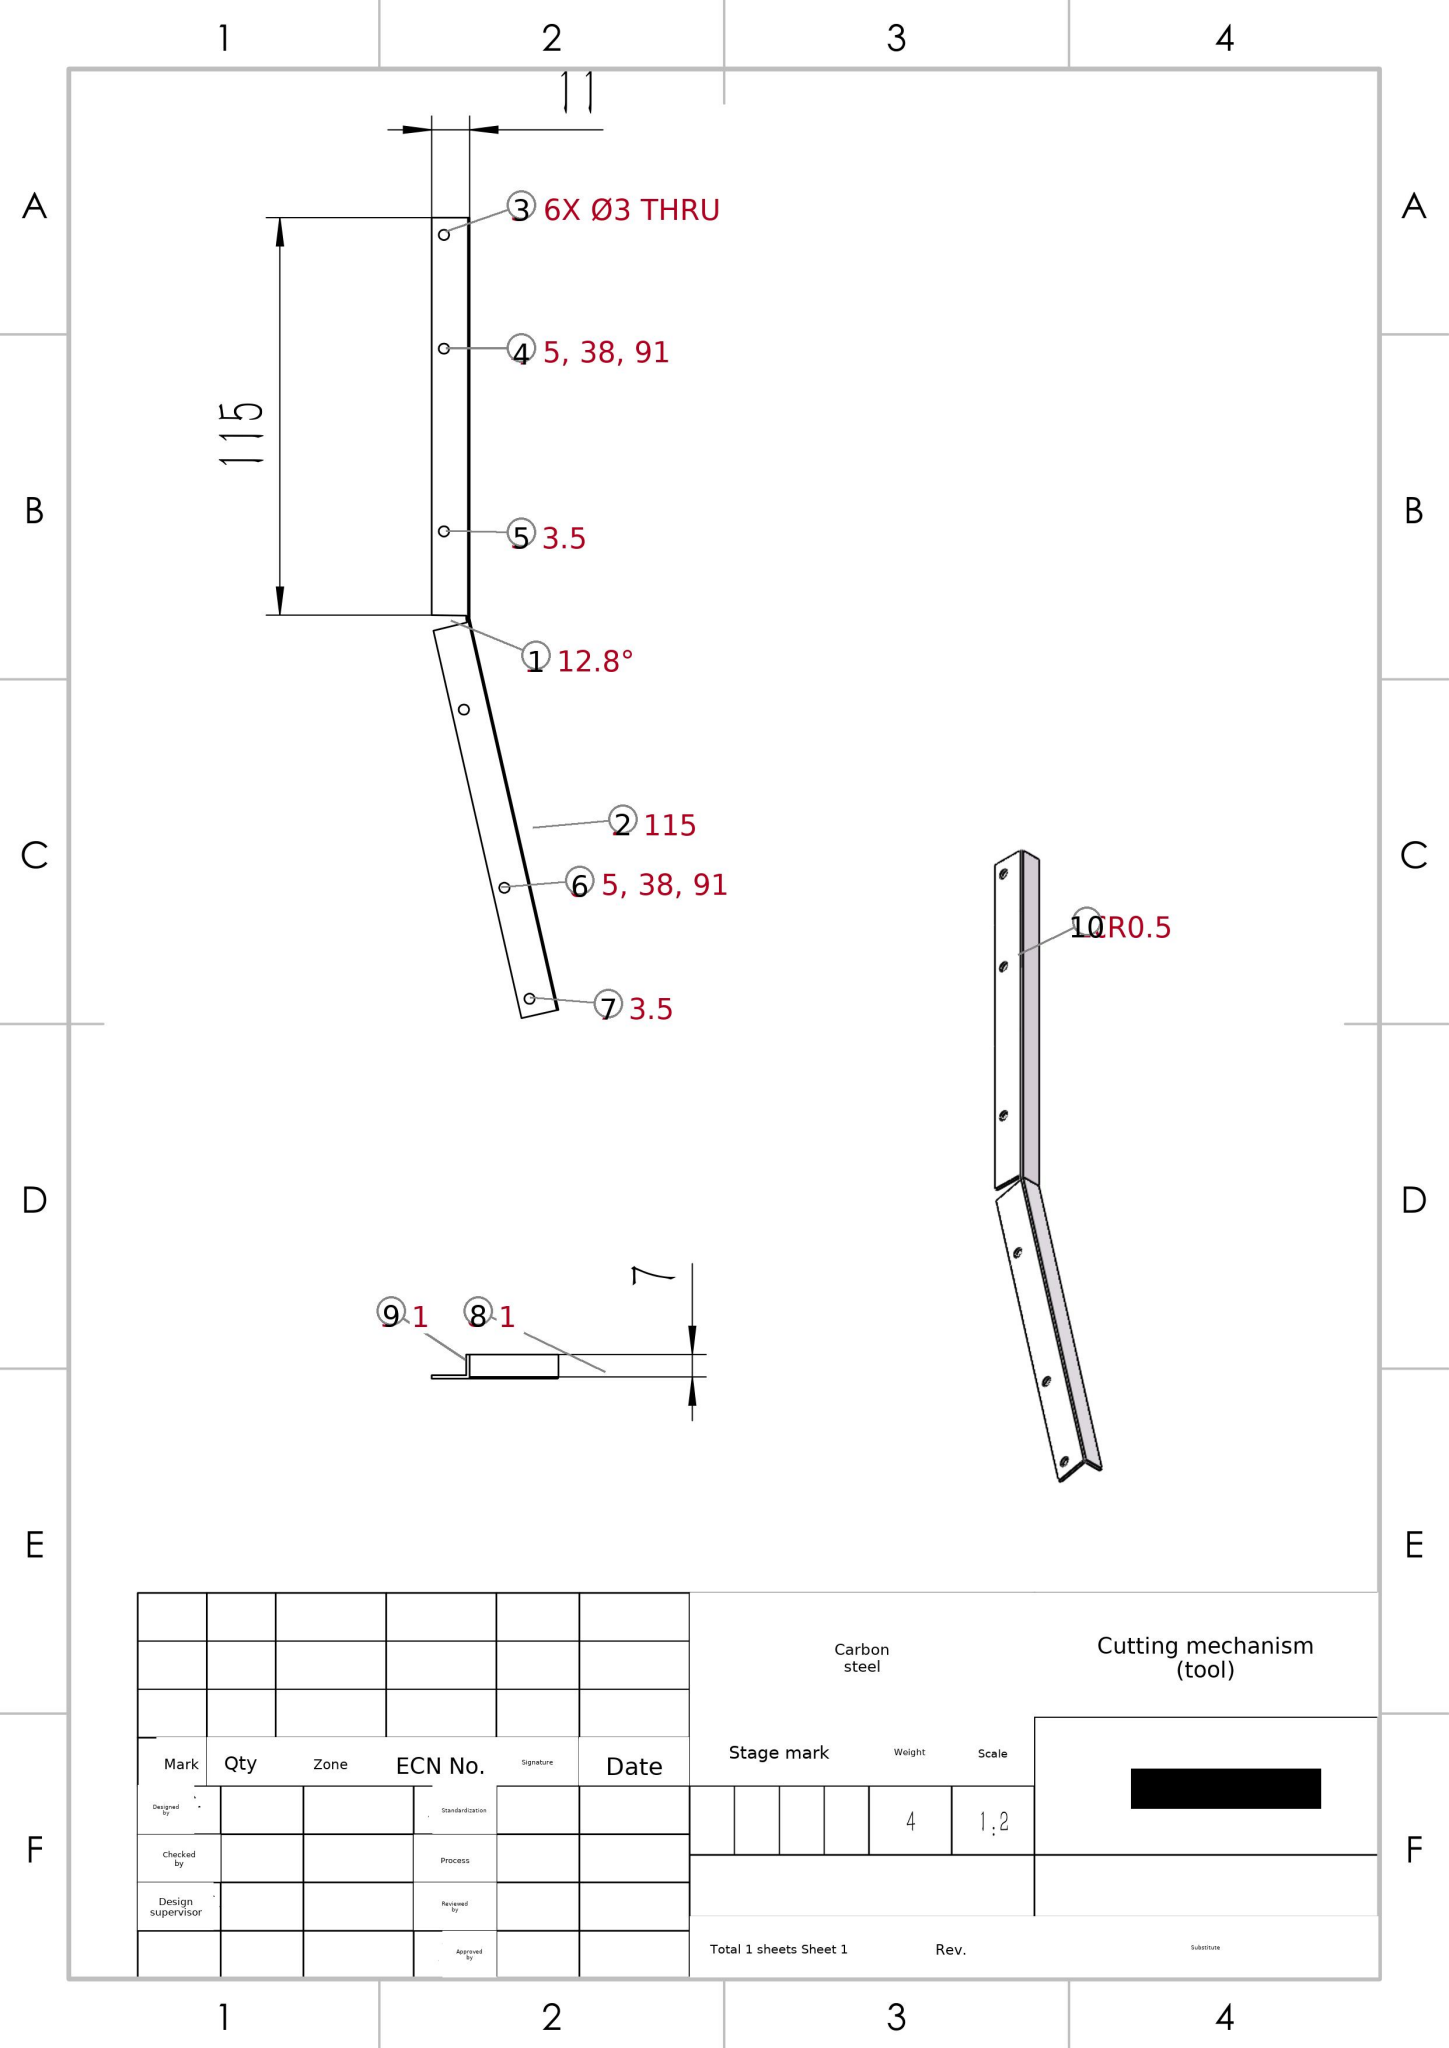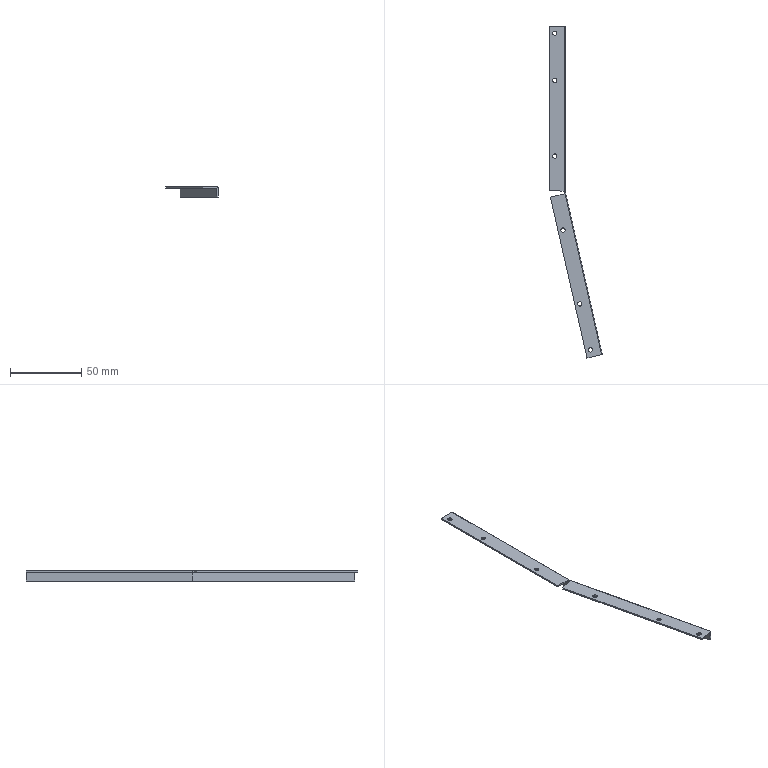Part | SolidWorks | mm | material Carbon steel | 1 solid | 28 faces | box 36.75 x 232.22 x 7 mm | volume 3882 mm3 | plane 14 | cylinder 14 | commonest cylinder face diameters 3 x12 1 x2
STEP:
#1=CARTESIAN_POINT('',(-10.,1.143,0.));
#2=VERTEX_POINT('',#1);
#3=CARTESIAN_POINT('',(0.,1.,0.));
#4=VERTEX_POINT('',#3);
#5=CARTESIAN_POINT('',(0.2085,0.997,-0.));
#6=DIRECTION('',(0.9999,-0.01434,-0.));
#7=VECTOR('',#6,1000.);
#8=LINE('',#5,#7);
#9=EDGE_CURVE('',#2,#4,#8,.T.);
#10=ORIENTED_EDGE('',*,*,#9,.T.);
#11=CARTESIAN_POINT('',(0.,1.,1.));
#12=VERTEX_POINT('',#11);
#13=CARTESIAN_POINT('',(0.,1.,-9.));
#14=DIRECTION('',(0.,0.,1.));
#15=VECTOR('',#14,1000.);
#16=LINE('',#13,#15);
#17=EDGE_CURVE('',#4,#12,#16,.T.);
#18=ORIENTED_EDGE('',*,*,#17,.T.);
#19=CARTESIAN_POINT('',(-10.,1.143,1.));
#20=VERTEX_POINT('',#19);
#21=CARTESIAN_POINT('',(0.01434,0.9998,1.));
#22=DIRECTION('',(-0.9999,0.01434,0.));
#23=VECTOR('',#22,1000.);
#24=LINE('',#21,#23);
#25=EDGE_CURVE('',#12,#20,#24,.T.);
#26=ORIENTED_EDGE('',*,*,#25,.T.);
#27=CARTESIAN_POINT('',(-10.,1.143,0.));
#28=DIRECTION('',(0.,0.,-1.));
#29=VECTOR('',#28,1000.);
#30=LINE('',#27,#29);
#31=EDGE_CURVE('',#20,#2,#30,.T.);
#32=ORIENTED_EDGE('',*,*,#31,.T.);
#33=EDGE_LOOP('',(#10,#18,#26,#32));
#34=FACE_OUTER_BOUND('',#33,.T.);
#35=CARTESIAN_POINT('',(0.01434,0.9998,-9.));
#36=DIRECTION('',(0.01434,0.9999,0.));
#37=DIRECTION('',(0.,0.,-1.));
#38=AXIS2_PLACEMENT_3D('',#35,#36,#37);
#39=PLANE('',#38);
#40=ADVANCED_FACE('',(#34),#39,.F.);
#41=CARTESIAN_POINT('',(-9.499,-3.329,1.));
#42=VERTEX_POINT('',#41);
#43=CARTESIAN_POINT('',(0.2214,-0.9752,1.));
#44=VERTEX_POINT('',#43);
#45=CARTESIAN_POINT('',(-12.308,-4.009,1.));
#46=DIRECTION('',(0.9719,0.2353,0.));
#47=VECTOR('',#46,1000.);
#48=LINE('',#45,#47);
#49=EDGE_CURVE('',#42,#44,#48,.T.);
#50=ORIENTED_EDGE('',*,*,#49,.T.);
#51=CARTESIAN_POINT('',(0.2214,-0.9752,0.));
#52=VERTEX_POINT('',#51);
#53=CARTESIAN_POINT('',(0.2214,-0.9752,-9.));
#54=DIRECTION('',(0.,0.,1.));
#55=VECTOR('',#54,1000.);
#56=LINE('',#53,#55);
#57=EDGE_CURVE('',#52,#44,#56,.T.);
#58=ORIENTED_EDGE('',*,*,#57,.F.);
#59=CARTESIAN_POINT('',(-9.499,-3.329,0.));
#60=VERTEX_POINT('',#59);
#61=CARTESIAN_POINT('',(-2.862,-1.722,0.));
#62=DIRECTION('',(-0.9719,-0.2353,0.));
#63=VECTOR('',#62,1000.);
#64=LINE('',#61,#63);
#65=EDGE_CURVE('',#52,#60,#64,.T.);
#66=ORIENTED_EDGE('',*,*,#65,.T.);
#67=CARTESIAN_POINT('',(-9.499,-3.329,0.));
#68=DIRECTION('',(0.,0.,-1.));
#69=VECTOR('',#68,1000.);
#70=LINE('',#67,#69);
#71=EDGE_CURVE('',#42,#60,#70,.T.);
#72=ORIENTED_EDGE('',*,*,#71,.F.);
#73=EDGE_LOOP('',(#50,#58,#66,#72));
#74=FACE_OUTER_BOUND('',#73,.T.);
#75=CARTESIAN_POINT('',(0.2353,-0.9718,-9.));
#76=DIRECTION('',(0.2353,-0.9719,0.));
#77=DIRECTION('',(0.,0.,-1.));
#78=AXIS2_PLACEMENT_3D('',#75,#76,#77);
#79=PLANE('',#78);
#80=ADVANCED_FACE('',(#74),#79,.F.);
#81=CARTESIAN_POINT('',(-7.96,25.45,0.));
#82=VERTEX_POINT('',#81);
#83=CARTESIAN_POINT('',(-7.96,25.45,1.));
#84=VERTEX_POINT('',#83);
#85=CARTESIAN_POINT('',(-7.96,25.45,-9.));
#86=DIRECTION('',(0.,0.,1.));
#87=VECTOR('',#86,1000.);
#88=LINE('',#85,#87);
#89=EDGE_CURVE('',#82,#84,#88,.T.);
#90=ORIENTED_EDGE('',*,*,#89,.F.);
#91=CARTESIAN_POINT('',(-4.96,25.45,-0.));
#92=VERTEX_POINT('',#91);
#93=CARTESIAN_POINT('',(-6.46,25.45,0.));
#94=DIRECTION('',(-0.,-0.,-1.));
#95=DIRECTION('',(-1.,0.,0.));
#96=AXIS2_PLACEMENT_3D('',#93,#94,#95);
#97=CIRCLE('',#96,1.5);
#98=EDGE_CURVE('',#82,#92,#97,.T.);
#99=ORIENTED_EDGE('',*,*,#98,.T.);
#100=CARTESIAN_POINT('',(-4.96,25.45,1.));
#101=VERTEX_POINT('',#100);
#102=CARTESIAN_POINT('',(-4.96,25.45,-9.));
#103=DIRECTION('',(0.,0.,1.));
#104=VECTOR('',#103,1000.);
#105=LINE('',#102,#104);
#106=EDGE_CURVE('',#92,#101,#105,.T.);
#107=ORIENTED_EDGE('',*,*,#106,.T.);
#108=CARTESIAN_POINT('',(-6.46,25.45,1.));
#109=DIRECTION('',(0.,0.,1.));
#110=DIRECTION('',(1.,0.,0.));
#111=AXIS2_PLACEMENT_3D('',#108,#109,#110);
#112=CIRCLE('',#111,1.5);
#113=EDGE_CURVE('',#101,#84,#112,.T.);
#114=ORIENTED_EDGE('',*,*,#113,.T.);
#115=EDGE_LOOP('',(#90,#99,#107,#114));
#116=FACE_OUTER_BOUND('',#115,.T.);
#117=CARTESIAN_POINT('',(-6.46,25.45,-9.));
#118=DIRECTION('',(0.,0.,1.));
#119=DIRECTION('',(1.,0.,0.));
#120=AXIS2_PLACEMENT_3D('',#117,#118,#119);
#121=CYLINDRICAL_SURFACE('',#120,1.5);
#122=ADVANCED_FACE('',(#116),#121,.F.);
#123=CARTESIAN_POINT('',(16.871,-110.115,-0.));
#124=VERTEX_POINT('',#123);
#125=CARTESIAN_POINT('',(16.871,-110.115,1.));
#126=VERTEX_POINT('',#125);
#127=CARTESIAN_POINT('',(16.871,-110.115,-9.));
#128=DIRECTION('',(0.,0.,1.));
#129=VECTOR('',#128,1000.);
#130=LINE('',#127,#129);
#131=EDGE_CURVE('',#124,#126,#130,.T.);
#132=ORIENTED_EDGE('',*,*,#131,.F.);
#133=CARTESIAN_POINT('',(19.871,-110.115,-0.));
#134=VERTEX_POINT('',#133);
#135=CARTESIAN_POINT('',(18.371,-110.115,-0.));
#136=DIRECTION('',(-0.,-0.,-1.));
#137=DIRECTION('',(-1.,0.,0.));
#138=AXIS2_PLACEMENT_3D('',#135,#136,#137);
#139=CIRCLE('',#138,1.5);
#140=EDGE_CURVE('',#124,#134,#139,.T.);
#141=ORIENTED_EDGE('',*,*,#140,.T.);
#142=CARTESIAN_POINT('',(19.871,-110.115,1.));
#143=VERTEX_POINT('',#142);
#144=CARTESIAN_POINT('',(19.871,-110.115,-9.));
#145=DIRECTION('',(0.,0.,1.));
#146=VECTOR('',#145,1000.);
#147=LINE('',#144,#146);
#148=EDGE_CURVE('',#134,#143,#147,.T.);
#149=ORIENTED_EDGE('',*,*,#148,.T.);
#150=CARTESIAN_POINT('',(18.371,-110.115,1.));
#151=DIRECTION('',(0.,0.,1.));
#152=DIRECTION('',(-1.,0.,0.));
#153=AXIS2_PLACEMENT_3D('',#150,#151,#152);
#154=CIRCLE('',#153,1.5);
#155=EDGE_CURVE('',#143,#126,#154,.T.);
#156=ORIENTED_EDGE('',*,*,#155,.T.);
#157=EDGE_LOOP('',(#132,#141,#149,#156));
#158=FACE_OUTER_BOUND('',#157,.T.);
#159=CARTESIAN_POINT('',(18.371,-110.115,-9.));
#160=DIRECTION('',(0.,0.,1.));
#161=DIRECTION('',(1.,0.,0.));
#162=AXIS2_PLACEMENT_3D('',#159,#160,#161);
#163=CYLINDRICAL_SURFACE('',#162,1.5);
#164=ADVANCED_FACE('',(#158),#163,.F.);
#165=CARTESIAN_POINT('',(9.566,-77.934,-0.));
#166=VERTEX_POINT('',#165);
#167=CARTESIAN_POINT('',(9.566,-77.934,1.));
#168=VERTEX_POINT('',#167);
#169=CARTESIAN_POINT('',(9.566,-77.934,-9.));
#170=DIRECTION('',(0.,0.,1.));
#171=VECTOR('',#170,1000.);
#172=LINE('',#169,#171);
#173=EDGE_CURVE('',#166,#168,#172,.T.);
#174=ORIENTED_EDGE('',*,*,#173,.F.);
#175=CARTESIAN_POINT('',(12.566,-77.934,-0.));
#176=VERTEX_POINT('',#175);
#177=CARTESIAN_POINT('',(11.066,-77.934,-0.));
#178=DIRECTION('',(-0.,-0.,-1.));
#179=DIRECTION('',(-1.,0.,0.));
#180=AXIS2_PLACEMENT_3D('',#177,#178,#179);
#181=CIRCLE('',#180,1.5);
#182=EDGE_CURVE('',#166,#176,#181,.T.);
#183=ORIENTED_EDGE('',*,*,#182,.T.);
#184=CARTESIAN_POINT('',(12.566,-77.934,1.));
#185=VERTEX_POINT('',#184);
#186=CARTESIAN_POINT('',(12.566,-77.934,-9.));
#187=DIRECTION('',(0.,0.,1.));
#188=VECTOR('',#187,1000.);
#189=LINE('',#186,#188);
#190=EDGE_CURVE('',#176,#185,#189,.T.);
#191=ORIENTED_EDGE('',*,*,#190,.T.);
#192=CARTESIAN_POINT('',(11.066,-77.934,1.));
#193=DIRECTION('',(0.,0.,1.));
#194=DIRECTION('',(-1.,0.,0.));
#195=AXIS2_PLACEMENT_3D('',#192,#193,#194);
#196=CIRCLE('',#195,1.5);
#197=EDGE_CURVE('',#185,#168,#196,.T.);
#198=ORIENTED_EDGE('',*,*,#197,.T.);
#199=EDGE_LOOP('',(#174,#183,#191,#198));
#200=FACE_OUTER_BOUND('',#199,.T.);
#201=CARTESIAN_POINT('',(11.066,-77.934,-9.));
#202=DIRECTION('',(0.,0.,1.));
#203=DIRECTION('',(1.,0.,0.));
#204=AXIS2_PLACEMENT_3D('',#201,#202,#203);
#205=CYLINDRICAL_SURFACE('',#204,1.5);
#206=ADVANCED_FACE('',(#200),#205,.F.);
#207=CARTESIAN_POINT('',(-2.166,-26.249,0.));
#208=VERTEX_POINT('',#207);
#209=CARTESIAN_POINT('',(-2.166,-26.249,1.));
#210=VERTEX_POINT('',#209);
#211=CARTESIAN_POINT('',(-2.166,-26.249,-9.));
#212=DIRECTION('',(0.,0.,1.));
#213=VECTOR('',#212,1000.);
#214=LINE('',#211,#213);
#215=EDGE_CURVE('',#208,#210,#214,.T.);
#216=ORIENTED_EDGE('',*,*,#215,.F.);
#217=CARTESIAN_POINT('',(0.8338,-26.249,-0.));
#218=VERTEX_POINT('',#217);
#219=CARTESIAN_POINT('',(-0.6662,-26.249,0.));
#220=DIRECTION('',(-0.,-0.,-1.));
#221=DIRECTION('',(-1.,0.,0.));
#222=AXIS2_PLACEMENT_3D('',#219,#220,#221);
#223=CIRCLE('',#222,1.5);
#224=EDGE_CURVE('',#208,#218,#223,.T.);
#225=ORIENTED_EDGE('',*,*,#224,.T.);
#226=CARTESIAN_POINT('',(0.8338,-26.249,1.));
#227=VERTEX_POINT('',#226);
#228=CARTESIAN_POINT('',(0.8338,-26.249,-9.));
#229=DIRECTION('',(0.,0.,1.));
#230=VECTOR('',#229,1000.);
#231=LINE('',#228,#230);
#232=EDGE_CURVE('',#218,#227,#231,.T.);
#233=ORIENTED_EDGE('',*,*,#232,.T.);
#234=CARTESIAN_POINT('',(-0.6662,-26.249,1.));
#235=DIRECTION('',(0.,0.,1.));
#236=DIRECTION('',(-1.,0.,0.));
#237=AXIS2_PLACEMENT_3D('',#234,#235,#236);
#238=CIRCLE('',#237,1.5);
#239=EDGE_CURVE('',#227,#210,#238,.T.);
#240=ORIENTED_EDGE('',*,*,#239,.T.);
#241=EDGE_LOOP('',(#216,#225,#233,#240));
#242=FACE_OUTER_BOUND('',#241,.T.);
#243=CARTESIAN_POINT('',(-0.6662,-26.249,-9.));
#244=DIRECTION('',(0.,0.,1.));
#245=DIRECTION('',(1.,0.,0.));
#246=AXIS2_PLACEMENT_3D('',#243,#244,#245);
#247=CYLINDRICAL_SURFACE('',#246,1.5);
#248=ADVANCED_FACE('',(#242),#247,.F.);
#249=CARTESIAN_POINT('',(-7.96,78.45,0.));
#250=VERTEX_POINT('',#249);
#251=CARTESIAN_POINT('',(-7.96,78.45,1.));
#252=VERTEX_POINT('',#251);
#253=CARTESIAN_POINT('',(-7.96,78.45,-9.));
#254=DIRECTION('',(0.,0.,1.));
#255=VECTOR('',#254,1000.);
#256=LINE('',#253,#255);
#257=EDGE_CURVE('',#250,#252,#256,.T.);
#258=ORIENTED_EDGE('',*,*,#257,.F.);
#259=CARTESIAN_POINT('',(-4.96,78.45,-0.));
#260=VERTEX_POINT('',#259);
#261=CARTESIAN_POINT('',(-6.46,78.45,0.));
#262=DIRECTION('',(-0.,-0.,-1.));
#263=DIRECTION('',(-1.,0.,0.));
#264=AXIS2_PLACEMENT_3D('',#261,#262,#263);
#265=CIRCLE('',#264,1.5);
#266=EDGE_CURVE('',#250,#260,#265,.T.);
#267=ORIENTED_EDGE('',*,*,#266,.T.);
#268=CARTESIAN_POINT('',(-4.96,78.45,1.));
#269=VERTEX_POINT('',#268);
#270=CARTESIAN_POINT('',(-4.96,78.45,-9.));
#271=DIRECTION('',(0.,0.,1.));
#272=VECTOR('',#271,1000.);
#273=LINE('',#270,#272);
#274=EDGE_CURVE('',#260,#269,#273,.T.);
#275=ORIENTED_EDGE('',*,*,#274,.T.);
#276=CARTESIAN_POINT('',(-6.46,78.45,1.));
#277=DIRECTION('',(0.,0.,1.));
#278=DIRECTION('',(1.,0.,0.));
#279=AXIS2_PLACEMENT_3D('',#276,#277,#278);
#280=CIRCLE('',#279,1.5);
#281=EDGE_CURVE('',#269,#252,#280,.T.);
#282=ORIENTED_EDGE('',*,*,#281,.T.);
#283=EDGE_LOOP('',(#258,#267,#275,#282));
#284=FACE_OUTER_BOUND('',#283,.T.);
#285=CARTESIAN_POINT('',(-6.46,78.45,-9.));
#286=DIRECTION('',(0.,0.,1.));
#287=DIRECTION('',(1.,0.,0.));
#288=AXIS2_PLACEMENT_3D('',#285,#286,#287);
#289=CYLINDRICAL_SURFACE('',#288,1.5);
#290=ADVANCED_FACE('',(#284),#289,.F.);
#291=CARTESIAN_POINT('',(-7.96,111.45,0.));
#292=VERTEX_POINT('',#291);
#293=CARTESIAN_POINT('',(-7.96,111.45,1.));
#294=VERTEX_POINT('',#293);
#295=CARTESIAN_POINT('',(-7.96,111.45,-9.));
#296=DIRECTION('',(0.,0.,1.));
#297=VECTOR('',#296,1000.);
#298=LINE('',#295,#297);
#299=EDGE_CURVE('',#292,#294,#298,.T.);
#300=ORIENTED_EDGE('',*,*,#299,.F.);
#301=CARTESIAN_POINT('',(-4.96,111.45,-0.));
#302=VERTEX_POINT('',#301);
#303=CARTESIAN_POINT('',(-6.46,111.45,0.));
#304=DIRECTION('',(-0.,-0.,-1.));
#305=DIRECTION('',(-1.,0.,0.));
#306=AXIS2_PLACEMENT_3D('',#303,#304,#305);
#307=CIRCLE('',#306,1.5);
#308=EDGE_CURVE('',#292,#302,#307,.T.);
#309=ORIENTED_EDGE('',*,*,#308,.T.);
#310=CARTESIAN_POINT('',(-4.96,111.45,1.));
#311=VERTEX_POINT('',#310);
#312=CARTESIAN_POINT('',(-4.96,111.45,-9.));
#313=DIRECTION('',(0.,0.,1.));
#314=VECTOR('',#313,1000.);
#315=LINE('',#312,#314);
#316=EDGE_CURVE('',#302,#311,#315,.T.);
#317=ORIENTED_EDGE('',*,*,#316,.T.);
#318=CARTESIAN_POINT('',(-6.46,111.45,1.));
#319=DIRECTION('',(0.,0.,1.));
#320=DIRECTION('',(1.,0.,0.));
#321=AXIS2_PLACEMENT_3D('',#318,#319,#320);
#322=CIRCLE('',#321,1.5);
#323=EDGE_CURVE('',#311,#294,#322,.T.);
#324=ORIENTED_EDGE('',*,*,#323,.T.);
#325=EDGE_LOOP('',(#300,#309,#317,#324));
#326=FACE_OUTER_BOUND('',#325,.T.);
#327=CARTESIAN_POINT('',(-6.46,111.45,-9.));
#328=DIRECTION('',(0.,0.,1.));
#329=DIRECTION('',(1.,0.,0.));
#330=AXIS2_PLACEMENT_3D('',#327,#328,#329);
#331=CYLINDRICAL_SURFACE('',#330,1.5);
#332=ADVANCED_FACE('',(#326),#331,.F.);
#333=CARTESIAN_POINT('',(26.752,-113.34,0.5));
#334=VERTEX_POINT('',#333);
#335=CARTESIAN_POINT('',(26.265,-113.451,1.));
#336=VERTEX_POINT('',#335);
#337=CARTESIAN_POINT('',(26.265,-113.451,0.5));
#338=DIRECTION('',(0.2214,-0.9752,0.));
#339=DIRECTION('',(0.9752,0.2214,0.));
#340=AXIS2_PLACEMENT_3D('',#337,#338,#339);
#341=CIRCLE('',#340,0.5);
#342=EDGE_CURVE('',#334,#336,#341,.T.);
#343=ORIENTED_EDGE('',*,*,#342,.T.);
#344=CARTESIAN_POINT('',(16.025,-115.775,1.));
#345=VERTEX_POINT('',#344);
#346=CARTESIAN_POINT('',(14.684,-116.079,1.));
#347=DIRECTION('',(-0.9752,-0.2214,0.));
#348=VECTOR('',#347,1000.);
#349=LINE('',#346,#348);
#350=EDGE_CURVE('',#336,#345,#349,.T.);
#351=ORIENTED_EDGE('',*,*,#350,.T.);
#352=CARTESIAN_POINT('',(16.025,-115.775,0.));
#353=VERTEX_POINT('',#352);
#354=CARTESIAN_POINT('',(16.025,-115.775,0.));
#355=DIRECTION('',(0.,0.,-1.));
#356=VECTOR('',#355,1000.);
#357=LINE('',#354,#356);
#358=EDGE_CURVE('',#345,#353,#357,.T.);
#359=ORIENTED_EDGE('',*,*,#358,.T.);
#360=CARTESIAN_POINT('',(25.777,-113.561,0.));
#361=VERTEX_POINT('',#360);
#362=CARTESIAN_POINT('',(24.315,-113.893,0.));
#363=DIRECTION('',(0.9752,0.2214,-0.));
#364=VECTOR('',#363,1000.);
#365=LINE('',#362,#364);
#366=EDGE_CURVE('',#353,#361,#365,.T.);
#367=ORIENTED_EDGE('',*,*,#366,.T.);
#368=CARTESIAN_POINT('',(25.777,-113.561,-6.));
#369=VERTEX_POINT('',#368);
#370=CARTESIAN_POINT('',(25.777,-113.561,-6.));
#371=DIRECTION('',(0.,0.,-1.));
#372=VECTOR('',#371,1000.);
#373=LINE('',#370,#372);
#374=EDGE_CURVE('',#361,#369,#373,.T.);
#375=ORIENTED_EDGE('',*,*,#374,.T.);
#376=CARTESIAN_POINT('',(26.752,-113.34,-6.));
#377=VERTEX_POINT('',#376);
#378=CARTESIAN_POINT('',(25.279,-113.674,-6.));
#379=DIRECTION('',(0.9752,0.2214,0.));
#380=VECTOR('',#379,1000.);
#381=LINE('',#378,#380);
#382=EDGE_CURVE('',#369,#377,#381,.T.);
#383=ORIENTED_EDGE('',*,*,#382,.T.);
#384=CARTESIAN_POINT('',(26.752,-113.34,0.5));
#385=DIRECTION('',(-0.,-0.,1.));
#386=VECTOR('',#385,1000.);
#387=LINE('',#384,#386);
#388=EDGE_CURVE('',#377,#334,#387,.T.);
#389=ORIENTED_EDGE('',*,*,#388,.T.);
#390=EDGE_LOOP('',(#343,#351,#359,#367,#375,#383,#389));
#391=FACE_OUTER_BOUND('',#390,.T.);
#392=CARTESIAN_POINT('',(21.389,-114.557,-2.5));
#393=DIRECTION('',(0.2214,-0.9752,0.));
#394=DIRECTION('',(0.,0.,-1.));
#395=AXIS2_PLACEMENT_3D('',#392,#393,#394);
#396=PLANE('',#395);
#397=ADVANCED_FACE('',(#391),#396,.T.);
#398=CARTESIAN_POINT('',(1.,0.1121,0.5));
#399=VERTEX_POINT('',#398);
#400=CARTESIAN_POINT('',(1.,116.45,0.5));
#401=VERTEX_POINT('',#400);
#402=CARTESIAN_POINT('',(1.,-13.543,0.5));
#403=DIRECTION('',(-0.,1.,0.));
#404=VECTOR('',#403,1000.);
#405=LINE('',#402,#404);
#406=EDGE_CURVE('',#399,#401,#405,.T.);
#407=ORIENTED_EDGE('',*,*,#406,.F.);
#408=CARTESIAN_POINT('',(1.,0.1121,-6.));
#409=VERTEX_POINT('',#408);
#410=CARTESIAN_POINT('',(1.,0.1121,0.5));
#411=DIRECTION('',(0.,0.,-1.));
#412=VECTOR('',#411,1000.);
#413=LINE('',#410,#412);
#414=EDGE_CURVE('',#399,#409,#413,.T.);
#415=ORIENTED_EDGE('',*,*,#414,.T.);
#416=CARTESIAN_POINT('',(1.,116.45,-6.));
#417=VERTEX_POINT('',#416);
#418=CARTESIAN_POINT('',(1.,-13.543,-6.));
#419=DIRECTION('',(-0.,1.,0.));
#420=VECTOR('',#419,1000.);
#421=LINE('',#418,#420);
#422=EDGE_CURVE('',#409,#417,#421,.T.);
#423=ORIENTED_EDGE('',*,*,#422,.T.);
#424=CARTESIAN_POINT('',(1.,116.45,0.5));
#425=DIRECTION('',(0.,0.,-1.));
#426=VECTOR('',#425,1000.);
#427=LINE('',#424,#426);
#428=EDGE_CURVE('',#401,#417,#427,.T.);
#429=ORIENTED_EDGE('',*,*,#428,.F.);
#430=EDGE_LOOP('',(#407,#415,#423,#429));
#431=FACE_OUTER_BOUND('',#430,.T.);
#432=CARTESIAN_POINT('',(1.,-13.543,0.5));
#433=DIRECTION('',(1.,0.,0.));
#434=DIRECTION('',(-0.,0.,1.));
#435=AXIS2_PLACEMENT_3D('',#432,#433,#434);
#436=PLANE('',#435);
#437=ADVANCED_FACE('',(#431),#436,.T.);
#438=CARTESIAN_POINT('',(0.5,0.05603,1.));
#439=VERTEX_POINT('',#438);
#440=CARTESIAN_POINT('',(0.5,116.45,1.));
#441=VERTEX_POINT('',#440);
#442=CARTESIAN_POINT('',(0.5,-13.543,1.));
#443=DIRECTION('',(-0.,1.,0.));
#444=VECTOR('',#443,1000.);
#445=LINE('',#442,#444);
#446=EDGE_CURVE('',#439,#441,#445,.T.);
#447=ORIENTED_EDGE('',*,*,#446,.F.);
#448=CARTESIAN_POINT('',(0.5,0.05603,1.));
#449=CARTESIAN_POINT('',(0.7929,0.08886,1.));
#450=CARTESIAN_POINT('',(1.,0.1121,0.7929));
#451=CARTESIAN_POINT('',(1.,0.1121,0.5));
#452=(BOUNDED_CURVE()B_SPLINE_CURVE(3,(#448,#449,#450,#451),.UNSPECIFIED.,.F.,.F.)B_SPLINE_CURVE_WITH_KNOTS((4,4),(4.712,6.283),.UNSPECIFIED.)CURVE()GEOMETRIC_REPRESENTATION_ITEM()RATIONAL_B_SPLINE_CURVE((1.,0.8047,0.8047,1.))REPRESENTATION_ITEM(''));
#453=EDGE_CURVE('',#439,#399,#452,.T.);
#454=ORIENTED_EDGE('',*,*,#453,.T.);
#455=ORIENTED_EDGE('',*,*,#406,.T.);
#456=CARTESIAN_POINT('',(0.5,116.45,0.5));
#457=DIRECTION('',(0.,1.,0.));
#458=DIRECTION('',(0.,0.,1.));
#459=AXIS2_PLACEMENT_3D('',#456,#457,#458);
#460=CIRCLE('',#459,0.5);
#461=EDGE_CURVE('',#441,#401,#460,.T.);
#462=ORIENTED_EDGE('',*,*,#461,.F.);
#463=EDGE_LOOP('',(#447,#454,#455,#462));
#464=FACE_OUTER_BOUND('',#463,.T.);
#465=CARTESIAN_POINT('',(0.5,-13.543,0.5));
#466=DIRECTION('',(0.,1.,0.));
#467=DIRECTION('',(-1.,0.,0.));
#468=AXIS2_PLACEMENT_3D('',#465,#466,#467);
#469=CYLINDRICAL_SURFACE('',#468,0.5);
#470=ADVANCED_FACE('',(#464),#469,.T.);
#471=ORIENTED_EDGE('',*,*,#323,.F.);
#472=CARTESIAN_POINT('',(-6.46,111.45,1.));
#473=DIRECTION('',(0.,0.,1.));
#474=DIRECTION('',(1.,0.,0.));
#475=AXIS2_PLACEMENT_3D('',#472,#473,#474);
#476=CIRCLE('',#475,1.5);
#477=EDGE_CURVE('',#294,#311,#476,.T.);
#478=ORIENTED_EDGE('',*,*,#477,.F.);
#479=EDGE_LOOP('',(#471,#478));
#480=FACE_BOUND('',#479,.T.);
#481=ORIENTED_EDGE('',*,*,#281,.F.);
#482=CARTESIAN_POINT('',(-6.46,78.45,1.));
#483=DIRECTION('',(0.,0.,1.));
#484=DIRECTION('',(1.,0.,0.));
#485=AXIS2_PLACEMENT_3D('',#482,#483,#484);
#486=CIRCLE('',#485,1.5);
#487=EDGE_CURVE('',#252,#269,#486,.T.);
#488=ORIENTED_EDGE('',*,*,#487,.F.);
#489=EDGE_LOOP('',(#481,#488));
#490=FACE_BOUND('',#489,.T.);
#491=ORIENTED_EDGE('',*,*,#239,.F.);
#492=CARTESIAN_POINT('',(-0.6662,-26.249,1.));
#493=DIRECTION('',(0.,0.,1.));
#494=DIRECTION('',(-1.,0.,0.));
#495=AXIS2_PLACEMENT_3D('',#492,#493,#494);
#496=CIRCLE('',#495,1.5);
#497=EDGE_CURVE('',#210,#227,#496,.T.);
#498=ORIENTED_EDGE('',*,*,#497,.F.);
#499=EDGE_LOOP('',(#491,#498));
#500=FACE_BOUND('',#499,.T.);
#501=ORIENTED_EDGE('',*,*,#197,.F.);
#502=CARTESIAN_POINT('',(11.066,-77.934,1.));
#503=DIRECTION('',(0.,0.,1.));
#504=DIRECTION('',(-1.,0.,0.));
#505=AXIS2_PLACEMENT_3D('',#502,#503,#504);
#506=CIRCLE('',#505,1.5);
#507=EDGE_CURVE('',#168,#185,#506,.T.);
#508=ORIENTED_EDGE('',*,*,#507,.F.);
#509=EDGE_LOOP('',(#501,#508));
#510=FACE_BOUND('',#509,.T.);
#511=ORIENTED_EDGE('',*,*,#155,.F.);
#512=CARTESIAN_POINT('',(18.371,-110.115,1.));
#513=DIRECTION('',(0.,0.,1.));
#514=DIRECTION('',(-1.,0.,0.));
#515=AXIS2_PLACEMENT_3D('',#512,#513,#514);
#516=CIRCLE('',#515,1.5);
#517=EDGE_CURVE('',#126,#143,#516,.T.);
#518=ORIENTED_EDGE('',*,*,#517,.F.);
#519=EDGE_LOOP('',(#511,#518));
#520=FACE_BOUND('',#519,.T.);
#521=ORIENTED_EDGE('',*,*,#113,.F.);
#522=CARTESIAN_POINT('',(-6.46,25.45,1.));
#523=DIRECTION('',(0.,0.,1.));
#524=DIRECTION('',(1.,0.,0.));
#525=AXIS2_PLACEMENT_3D('',#522,#523,#524);
#526=CIRCLE('',#525,1.5);
#527=EDGE_CURVE('',#84,#101,#526,.T.);
#528=ORIENTED_EDGE('',*,*,#527,.F.);
#529=EDGE_LOOP('',(#521,#528));
#530=FACE_BOUND('',#529,.T.);
#531=ORIENTED_EDGE('',*,*,#25,.F.);
#532=CARTESIAN_POINT('',(0.,-0.,1.));
#533=VERTEX_POINT('',#532);
#534=CARTESIAN_POINT('',(0.,0.,1.));
#535=DIRECTION('',(0.,-1.,0.));
#536=VECTOR('',#535,1000.);
#537=LINE('',#534,#536);
#538=EDGE_CURVE('',#12,#533,#537,.T.);
#539=ORIENTED_EDGE('',*,*,#538,.T.);
#540=CARTESIAN_POINT('',(0.,0.,1.));
#541=DIRECTION('',(-0.2214,0.9752,0.));
#542=VECTOR('',#541,1000.);
#543=LINE('',#540,#542);
#544=EDGE_CURVE('',#44,#533,#543,.T.);
#545=ORIENTED_EDGE('',*,*,#544,.F.);
#546=ORIENTED_EDGE('',*,*,#49,.F.);
#547=CARTESIAN_POINT('',(-10.,-1.121,1.));
#548=DIRECTION('',(0.2214,-0.9752,0.));
#549=VECTOR('',#548,1000.);
#550=LINE('',#547,#549);
#551=EDGE_CURVE('',#42,#345,#550,.T.);
#552=ORIENTED_EDGE('',*,*,#551,.T.);
#553=ORIENTED_EDGE('',*,*,#350,.F.);
#554=CARTESIAN_POINT('',(0.5,0.05603,1.));
#555=DIRECTION('',(0.2214,-0.9752,0.));
#556=VECTOR('',#555,1000.);
#557=LINE('',#554,#556);
#558=EDGE_CURVE('',#439,#336,#557,.T.);
#559=ORIENTED_EDGE('',*,*,#558,.F.);
#560=ORIENTED_EDGE('',*,*,#446,.T.);
#561=CARTESIAN_POINT('',(-10.,116.45,1.));
#562=VERTEX_POINT('',#561);
#563=CARTESIAN_POINT('',(-10.,116.45,1.));
#564=DIRECTION('',(1.,0.,0.));
#565=VECTOR('',#564,1000.);
#566=LINE('',#563,#565);
#567=EDGE_CURVE('',#562,#441,#566,.T.);
#568=ORIENTED_EDGE('',*,*,#567,.F.);
#569=CARTESIAN_POINT('',(-10.,-13.543,1.));
#570=DIRECTION('',(-0.,1.,0.));
#571=VECTOR('',#570,1000.);
#572=LINE('',#569,#571);
#573=EDGE_CURVE('',#20,#562,#572,.T.);
#574=ORIENTED_EDGE('',*,*,#573,.F.);
#575=EDGE_LOOP('',(#531,#539,#545,#546,#552,#553,#559,#560,#568,#574));
#576=FACE_OUTER_BOUND('',#575,.T.);
#577=CARTESIAN_POINT('',(-10.,-13.543,1.));
#578=DIRECTION('',(0.,0.,1.));
#579=DIRECTION('',(1.,0.,0.));
#580=AXIS2_PLACEMENT_3D('',#577,#578,#579);
#581=PLANE('',#580);
#582=ADVANCED_FACE('',(#480,#490,#500,#510,#520,#530,#576),#581,.T.);
#583=ORIENTED_EDGE('',*,*,#31,.F.);
#584=ORIENTED_EDGE('',*,*,#573,.T.);
#585=CARTESIAN_POINT('',(-10.,116.45,0.));
#586=VERTEX_POINT('',#585);
#587=CARTESIAN_POINT('',(-10.,116.45,0.));
#588=DIRECTION('',(0.,0.,1.));
#589=VECTOR('',#588,1000.);
#590=LINE('',#587,#589);
#591=EDGE_CURVE('',#586,#562,#590,.T.);
#592=ORIENTED_EDGE('',*,*,#591,.F.);
#593=CARTESIAN_POINT('',(-10.,-13.543,0.));
#594=DIRECTION('',(-0.,1.,0.));
#595=VECTOR('',#594,1000.);
#596=LINE('',#593,#595);
#597=EDGE_CURVE('',#2,#586,#596,.T.);
#598=ORIENTED_EDGE('',*,*,#597,.F.);
#599=EDGE_LOOP('',(#583,#584,#592,#598));
#600=FACE_OUTER_BOUND('',#599,.T.);
#601=CARTESIAN_POINT('',(-10.,-13.543,0.));
#602=DIRECTION('',(-1.,-0.,0.));
#603=DIRECTION('',(-0.,1.,0.));
#604=AXIS2_PLACEMENT_3D('',#601,#602,#603);
#605=PLANE('',#604);
#606=ADVANCED_FACE('',(#600),#605,.T.);
#607=CARTESIAN_POINT('',(-0.6662,-26.249,0.));
#608=DIRECTION('',(-0.,-0.,-1.));
#609=DIRECTION('',(-1.,0.,0.));
#610=AXIS2_PLACEMENT_3D('',#607,#608,#609);
#611=CIRCLE('',#610,1.5);
#612=EDGE_CURVE('',#218,#208,#611,.T.);
#613=ORIENTED_EDGE('',*,*,#612,.F.);
#614=ORIENTED_EDGE('',*,*,#224,.F.);
#615=EDGE_LOOP('',(#613,#614));
#616=FACE_BOUND('',#615,.T.);
#617=CARTESIAN_POINT('',(11.066,-77.934,-0.));
#618=DIRECTION('',(-0.,-0.,-1.));
#619=DIRECTION('',(-1.,0.,0.));
#620=AXIS2_PLACEMENT_3D('',#617,#618,#619);
#621=CIRCLE('',#620,1.5);
#622=EDGE_CURVE('',#176,#166,#621,.T.);
#623=ORIENTED_EDGE('',*,*,#622,.F.);
#624=ORIENTED_EDGE('',*,*,#182,.F.);
#625=EDGE_LOOP('',(#623,#624));
#626=FACE_BOUND('',#625,.T.);
#627=CARTESIAN_POINT('',(18.371,-110.115,-0.));
#628=DIRECTION('',(-0.,-0.,-1.));
#629=DIRECTION('',(-1.,0.,0.));
#630=AXIS2_PLACEMENT_3D('',#627,#628,#629);
#631=CIRCLE('',#630,1.5);
#632=EDGE_CURVE('',#134,#124,#631,.T.);
#633=ORIENTED_EDGE('',*,*,#632,.F.);
#634=ORIENTED_EDGE('',*,*,#140,.F.);
#635=EDGE_LOOP('',(#633,#634));
#636=FACE_BOUND('',#635,.T.);
#637=ORIENTED_EDGE('',*,*,#65,.F.);
#638=CARTESIAN_POINT('',(0.,-0.,0.));
#639=DIRECTION('',(0.2214,-0.9752,0.));
#640=VECTOR('',#639,1000.);
#641=LINE('',#638,#640);
#642=EDGE_CURVE('',#52,#361,#641,.T.);
#643=ORIENTED_EDGE('',*,*,#642,.T.);
#644=ORIENTED_EDGE('',*,*,#366,.F.);
#645=CARTESIAN_POINT('',(-10.,-1.121,0.));
#646=DIRECTION('',(0.2214,-0.9752,0.));
#647=VECTOR('',#646,1000.);
#648=LINE('',#645,#647);
#649=EDGE_CURVE('',#60,#353,#648,.T.);
#650=ORIENTED_EDGE('',*,*,#649,.F.);
#651=EDGE_LOOP('',(#637,#643,#644,#650));
#652=FACE_OUTER_BOUND('',#651,.T.);
#653=CARTESIAN_POINT('',(0.,-13.543,0.));
#654=DIRECTION('',(-0.,-0.,-1.));
#655=DIRECTION('',(-1.,0.,0.));
#656=AXIS2_PLACEMENT_3D('',#653,#654,#655);
#657=PLANE('',#656);
#658=ADVANCED_FACE('',(#616,#626,#636,#652),#657,.T.);
#659=CARTESIAN_POINT('',(0.,116.45,-6.));
#660=VERTEX_POINT('',#659);
#661=CARTESIAN_POINT('',(0.,116.45,0.));
#662=VERTEX_POINT('',#661);
#663=CARTESIAN_POINT('',(0.,116.45,-6.));
#664=DIRECTION('',(-0.,0.,1.));
#665=VECTOR('',#664,1000.);
#666=LINE('',#663,#665);
#667=EDGE_CURVE('',#660,#662,#666,.T.);
#668=ORIENTED_EDGE('',*,*,#667,.F.);
#669=CARTESIAN_POINT('',(0.,-0.,-6.));
#670=VERTEX_POINT('',#669);
#671=CARTESIAN_POINT('',(0.,-13.543,-6.));
#672=DIRECTION('',(-0.,1.,0.));
#673=VECTOR('',#672,1000.);
#674=LINE('',#671,#673);
#675=EDGE_CURVE('',#670,#660,#674,.T.);
#676=ORIENTED_EDGE('',*,*,#675,.F.);
#677=CARTESIAN_POINT('',(0.,0.,-6.));
#678=DIRECTION('',(-0.,-0.,1.));
#679=VECTOR('',#678,1000.);
#680=LINE('',#677,#679);
#681=EDGE_CURVE('',#670,#533,#680,.T.);
#682=ORIENTED_EDGE('',*,*,#681,.T.);
#683=ORIENTED_EDGE('',*,*,#538,.F.);
#684=ORIENTED_EDGE('',*,*,#17,.F.);
#685=CARTESIAN_POINT('',(0.,-13.543,0.));
#686=DIRECTION('',(-0.,1.,0.));
#687=VECTOR('',#686,1000.);
#688=LINE('',#685,#687);
#689=EDGE_CURVE('',#4,#662,#688,.T.);
#690=ORIENTED_EDGE('',*,*,#689,.T.);
#691=EDGE_LOOP('',(#668,#676,#682,#683,#684,#690));
#692=FACE_OUTER_BOUND('',#691,.T.);
#693=CARTESIAN_POINT('',(0.,-13.543,-6.));
#694=DIRECTION('',(-1.,-0.,-0.));
#695=DIRECTION('',(-0.,0.,1.));
#696=AXIS2_PLACEMENT_3D('',#693,#694,#695);
#697=PLANE('',#696);
#698=ADVANCED_FACE('',(#692),#697,.T.);
#699=ORIENTED_EDGE('',*,*,#422,.F.);
#700=CARTESIAN_POINT('',(1.,0.1121,-6.));
#701=DIRECTION('',(0.2214,-0.9752,0.));
#702=VECTOR('',#701,1000.);
#703=LINE('',#700,#702);
#704=EDGE_CURVE('',#409,#377,#703,.T.);
#705=ORIENTED_EDGE('',*,*,#704,.T.);
#706=ORIENTED_EDGE('',*,*,#382,.F.);
#707=CARTESIAN_POINT('',(0.,-0.,-6.));
#708=DIRECTION('',(0.2214,-0.9752,0.));
#709=VECTOR('',#708,1000.);
#710=LINE('',#707,#709);
#711=EDGE_CURVE('',#670,#369,#710,.T.);
#712=ORIENTED_EDGE('',*,*,#711,.F.);
#713=ORIENTED_EDGE('',*,*,#675,.T.);
#714=CARTESIAN_POINT('',(1.,116.45,-6.));
#715=DIRECTION('',(-1.,0.,0.));
#716=VECTOR('',#715,1000.);
#717=LINE('',#714,#716);
#718=EDGE_CURVE('',#417,#660,#717,.T.);
#719=ORIENTED_EDGE('',*,*,#718,.F.);
#720=EDGE_LOOP('',(#699,#705,#706,#712,#713,#719));
#721=FACE_OUTER_BOUND('',#720,.T.);
#722=CARTESIAN_POINT('',(1.,-13.543,-6.));
#723=DIRECTION('',(0.,0.,-1.));
#724=DIRECTION('',(0.,-1.,0.));
#725=AXIS2_PLACEMENT_3D('',#722,#723,#724);
#726=PLANE('',#725);
#727=ADVANCED_FACE('',(#721),#726,.T.);
#728=ORIENTED_EDGE('',*,*,#718,.T.);
#729=ORIENTED_EDGE('',*,*,#667,.T.);
#730=CARTESIAN_POINT('',(0.,116.45,0.));
#731=DIRECTION('',(-1.,0.,0.));
#732=VECTOR('',#731,1000.);
#733=LINE('',#730,#732);
#734=EDGE_CURVE('',#662,#586,#733,.T.);
#735=ORIENTED_EDGE('',*,*,#734,.T.);
#736=ORIENTED_EDGE('',*,*,#591,.T.);
#737=ORIENTED_EDGE('',*,*,#567,.T.);
#738=ORIENTED_EDGE('',*,*,#461,.T.);
#739=ORIENTED_EDGE('',*,*,#428,.T.);
#740=EDGE_LOOP('',(#728,#729,#735,#736,#737,#738,#739));
#741=FACE_OUTER_BOUND('',#740,.T.);
#742=CARTESIAN_POINT('',(0.5,116.45,0.5));
#743=DIRECTION('',(0.,1.,0.));
#744=DIRECTION('',(1.,0.,0.));
#745=AXIS2_PLACEMENT_3D('',#742,#743,#744);
#746=PLANE('',#745);
#747=ADVANCED_FACE('',(#741),#746,.T.);
#748=ORIENTED_EDGE('',*,*,#551,.F.);
#749=ORIENTED_EDGE('',*,*,#71,.T.);
#750=ORIENTED_EDGE('',*,*,#649,.T.);
#751=ORIENTED_EDGE('',*,*,#358,.F.);
#752=EDGE_LOOP('',(#748,#749,#750,#751));
#753=FACE_OUTER_BOUND('',#752,.T.);
#754=CARTESIAN_POINT('',(-10.,-1.121,0.));
#755=DIRECTION('',(0.9752,0.2214,0.));
#756=DIRECTION('',(0.,0.,-1.));
#757=AXIS2_PLACEMENT_3D('',#754,#755,#756);
#758=PLANE('',#757);
#759=ADVANCED_FACE('',(#753),#758,.F.);
#760=ORIENTED_EDGE('',*,*,#642,.F.);
#761=ORIENTED_EDGE('',*,*,#57,.T.);
#762=ORIENTED_EDGE('',*,*,#544,.T.);
#763=ORIENTED_EDGE('',*,*,#681,.F.);
#764=ORIENTED_EDGE('',*,*,#711,.T.);
#765=ORIENTED_EDGE('',*,*,#374,.F.);
#766=EDGE_LOOP('',(#760,#761,#762,#763,#764,#765));
#767=FACE_OUTER_BOUND('',#766,.T.);
#768=CARTESIAN_POINT('',(0.,0.,-6.));
#769=DIRECTION('',(0.9752,0.2214,0.));
#770=DIRECTION('',(0.,0.,-1.));
#771=AXIS2_PLACEMENT_3D('',#768,#769,#770);
#772=PLANE('',#771);
#773=ADVANCED_FACE('',(#767),#772,.F.);
#774=ORIENTED_EDGE('',*,*,#388,.F.);
#775=ORIENTED_EDGE('',*,*,#704,.F.);
#776=ORIENTED_EDGE('',*,*,#414,.F.);
#777=CARTESIAN_POINT('',(1.,0.1121,0.5));
#778=DIRECTION('',(0.2214,-0.9752,0.));
#779=VECTOR('',#778,1000.);
#780=LINE('',#777,#779);
#781=EDGE_CURVE('',#399,#334,#780,.T.);
#782=ORIENTED_EDGE('',*,*,#781,.T.);
#783=EDGE_LOOP('',(#774,#775,#776,#782));
#784=FACE_OUTER_BOUND('',#783,.T.);
#785=CARTESIAN_POINT('',(1.,0.1121,0.5));
#786=DIRECTION('',(-0.9752,-0.2214,-0.));
#787=DIRECTION('',(-0.2214,0.9752,0.));
#788=AXIS2_PLACEMENT_3D('',#785,#786,#787);
#789=PLANE('',#788);
#790=ADVANCED_FACE('',(#784),#789,.F.);
#791=ORIENTED_EDGE('',*,*,#342,.F.);
#792=ORIENTED_EDGE('',*,*,#781,.F.);
#793=ORIENTED_EDGE('',*,*,#453,.F.);
#794=ORIENTED_EDGE('',*,*,#558,.T.);
#795=EDGE_LOOP('',(#791,#792,#793,#794));
#796=FACE_OUTER_BOUND('',#795,.T.);
#797=CARTESIAN_POINT('',(0.5,0.05603,0.5));
#798=DIRECTION('',(0.2214,-0.9752,0.));
#799=DIRECTION('',(0.9752,0.2214,0.));
#800=AXIS2_PLACEMENT_3D('',#797,#798,#799);
#801=CYLINDRICAL_SURFACE('',#800,0.5);
#802=ADVANCED_FACE('',(#796),#801,.T.);
#803=CARTESIAN_POINT('',(-6.46,25.45,0.));
#804=DIRECTION('',(-0.,-0.,-1.));
#805=DIRECTION('',(-1.,0.,0.));
#806=AXIS2_PLACEMENT_3D('',#803,#804,#805);
#807=CIRCLE('',#806,1.5);
#808=EDGE_CURVE('',#92,#82,#807,.T.);
#809=ORIENTED_EDGE('',*,*,#808,.F.);
#810=ORIENTED_EDGE('',*,*,#98,.F.);
#811=EDGE_LOOP('',(#809,#810));
#812=FACE_BOUND('',#811,.T.);
#813=CARTESIAN_POINT('',(-6.46,78.45,0.));
#814=DIRECTION('',(-0.,-0.,-1.));
#815=DIRECTION('',(-1.,0.,0.));
#816=AXIS2_PLACEMENT_3D('',#813,#814,#815);
#817=CIRCLE('',#816,1.5);
#818=EDGE_CURVE('',#260,#250,#817,.T.);
#819=ORIENTED_EDGE('',*,*,#818,.F.);
#820=ORIENTED_EDGE('',*,*,#266,.F.);
#821=EDGE_LOOP('',(#819,#820));
#822=FACE_BOUND('',#821,.T.);
#823=CARTESIAN_POINT('',(-6.46,111.45,0.));
#824=DIRECTION('',(-0.,-0.,-1.));
#825=DIRECTION('',(-1.,0.,0.));
#826=AXIS2_PLACEMENT_3D('',#823,#824,#825);
#827=CIRCLE('',#826,1.5);
#828=EDGE_CURVE('',#302,#292,#827,.T.);
#829=ORIENTED_EDGE('',*,*,#828,.F.);
#830=ORIENTED_EDGE('',*,*,#308,.F.);
#831=EDGE_LOOP('',(#829,#830));
#832=FACE_BOUND('',#831,.T.);
#833=ORIENTED_EDGE('',*,*,#9,.F.);
#834=ORIENTED_EDGE('',*,*,#597,.T.);
#835=ORIENTED_EDGE('',*,*,#734,.F.);
#836=ORIENTED_EDGE('',*,*,#689,.F.);
#837=EDGE_LOOP('',(#833,#834,#835,#836));
#838=FACE_OUTER_BOUND('',#837,.T.);
#839=CARTESIAN_POINT('',(0.,-13.543,0.));
#840=DIRECTION('',(-0.,-0.,-1.));
#841=DIRECTION('',(-1.,0.,0.));
#842=AXIS2_PLACEMENT_3D('',#839,#840,#841);
#843=PLANE('',#842);
#844=ADVANCED_FACE('',(#812,#822,#832,#838),#843,.T.);
#845=ORIENTED_EDGE('',*,*,#828,.T.);
#846=ORIENTED_EDGE('',*,*,#299,.T.);
#847=ORIENTED_EDGE('',*,*,#477,.T.);
#848=ORIENTED_EDGE('',*,*,#316,.F.);
#849=EDGE_LOOP('',(#845,#846,#847,#848));
#850=FACE_OUTER_BOUND('',#849,.T.);
#851=CARTESIAN_POINT('',(-6.46,111.45,-9.));
#852=DIRECTION('',(0.,0.,1.));
#853=DIRECTION('',(1.,0.,0.));
#854=AXIS2_PLACEMENT_3D('',#851,#852,#853);
#855=CYLINDRICAL_SURFACE('',#854,1.5);
#856=ADVANCED_FACE('',(#850),#855,.F.);
#857=ORIENTED_EDGE('',*,*,#818,.T.);
#858=ORIENTED_EDGE('',*,*,#257,.T.);
#859=ORIENTED_EDGE('',*,*,#487,.T.);
#860=ORIENTED_EDGE('',*,*,#274,.F.);
#861=EDGE_LOOP('',(#857,#858,#859,#860));
#862=FACE_OUTER_BOUND('',#861,.T.);
#863=CARTESIAN_POINT('',(-6.46,78.45,-9.));
#864=DIRECTION('',(0.,0.,1.));
#865=DIRECTION('',(1.,0.,0.));
#866=AXIS2_PLACEMENT_3D('',#863,#864,#865);
#867=CYLINDRICAL_SURFACE('',#866,1.5);
#868=ADVANCED_FACE('',(#862),#867,.F.);
#869=ORIENTED_EDGE('',*,*,#612,.T.);
#870=ORIENTED_EDGE('',*,*,#215,.T.);
#871=ORIENTED_EDGE('',*,*,#497,.T.);
#872=ORIENTED_EDGE('',*,*,#232,.F.);
#873=EDGE_LOOP('',(#869,#870,#871,#872));
#874=FACE_OUTER_BOUND('',#873,.T.);
#875=CARTESIAN_POINT('',(-0.6662,-26.249,-9.));
#876=DIRECTION('',(0.,0.,1.));
#877=DIRECTION('',(1.,0.,0.));
#878=AXIS2_PLACEMENT_3D('',#875,#876,#877);
#879=CYLINDRICAL_SURFACE('',#878,1.5);
#880=ADVANCED_FACE('',(#874),#879,.F.);
#881=ORIENTED_EDGE('',*,*,#622,.T.);
#882=ORIENTED_EDGE('',*,*,#173,.T.);
#883=ORIENTED_EDGE('',*,*,#507,.T.);
#884=ORIENTED_EDGE('',*,*,#190,.F.);
#885=EDGE_LOOP('',(#881,#882,#883,#884));
#886=FACE_OUTER_BOUND('',#885,.T.);
#887=CARTESIAN_POINT('',(11.066,-77.934,-9.));
#888=DIRECTION('',(0.,0.,1.));
#889=DIRECTION('',(1.,0.,0.));
#890=AXIS2_PLACEMENT_3D('',#887,#888,#889);
#891=CYLINDRICAL_SURFACE('',#890,1.5);
#892=ADVANCED_FACE('',(#886),#891,.F.);
#893=ORIENTED_EDGE('',*,*,#632,.T.);
#894=ORIENTED_EDGE('',*,*,#131,.T.);
#895=ORIENTED_EDGE('',*,*,#517,.T.);
#896=ORIENTED_EDGE('',*,*,#148,.F.);
#897=EDGE_LOOP('',(#893,#894,#895,#896));
#898=FACE_OUTER_BOUND('',#897,.T.);
#899=CARTESIAN_POINT('',(18.371,-110.115,-9.));
#900=DIRECTION('',(0.,0.,1.));
#901=DIRECTION('',(1.,0.,0.));
#902=AXIS2_PLACEMENT_3D('',#899,#900,#901);
#903=CYLINDRICAL_SURFACE('',#902,1.5);
#904=ADVANCED_FACE('',(#898),#903,.F.);
#905=ORIENTED_EDGE('',*,*,#808,.T.);
#906=ORIENTED_EDGE('',*,*,#89,.T.);
#907=ORIENTED_EDGE('',*,*,#527,.T.);
#908=ORIENTED_EDGE('',*,*,#106,.F.);
#909=EDGE_LOOP('',(#905,#906,#907,#908));
#910=FACE_OUTER_BOUND('',#909,.T.);
#911=CARTESIAN_POINT('',(-6.46,25.45,-9.));
#912=DIRECTION('',(0.,0.,1.));
#913=DIRECTION('',(1.,0.,0.));
#914=AXIS2_PLACEMENT_3D('',#911,#912,#913);
#915=CYLINDRICAL_SURFACE('',#914,1.5);
#916=ADVANCED_FACE('',(#910),#915,.F.);
#917=CLOSED_SHELL('',(#40,#80,#122,#164,#206,#248,#290,#332,#397,#437,#470,#582,#606,#658,#698,#727,#747,#759,#773,#790,#802,#844,#856,#868,#880,#892,#904,#916));
#918=MANIFOLD_SOLID_BREP('',#917);
#919=CARTESIAN_POINT('',(0.,0.,0.));
#920=DIRECTION('',(0.,0.,1.));
#921=DIRECTION('',(1.,0.,0.));
#922=AXIS2_PLACEMENT_3D('',#919,#920,#921);
#923=(LENGTH_UNIT()NAMED_UNIT(*)SI_UNIT(.MILLI.,.METRE.));
#924=UNCERTAINTY_MEASURE_WITH_UNIT(LENGTH_MEASURE(0.00001),#923,'','');
#925=(NAMED_UNIT(*)PLANE_ANGLE_UNIT()SI_UNIT($,.RADIAN.));
#926=(NAMED_UNIT(*)SI_UNIT($,.STERADIAN.)SOLID_ANGLE_UNIT());
#927=(GEOMETRIC_REPRESENTATION_CONTEXT(3)GLOBAL_UNCERTAINTY_ASSIGNED_CONTEXT((#924))GLOBAL_UNIT_ASSIGNED_CONTEXT((#923,#925,#926))REPRESENTATION_CONTEXT('',''));
#928=ADVANCED_BREP_SHAPE_REPRESENTATION('',(#918,#922),#927);